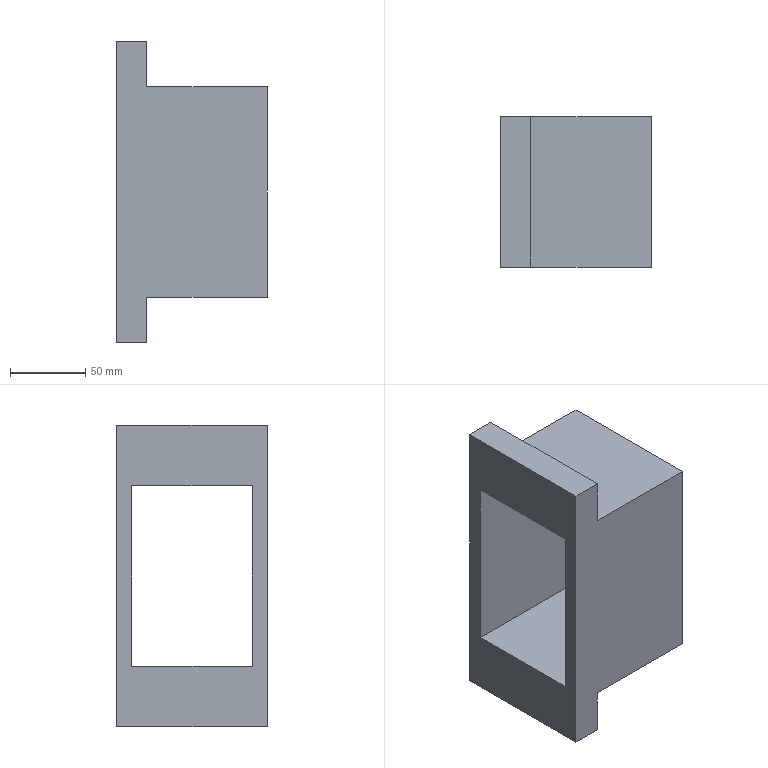Component | SolidWorks | ST60-03-1 | 1 solid | 14 faces | box 100 x 100 x 200 mm | volume 560000 mm3 | plane 14
build123d program:
from build123d import *

# Parameters (mm, degrees)
BOSS_EXTRUDE1_DEPTH = 100
SKETCH2_W           = 120
SKETCH2_H           = 80
CUT_EXTRUDE1_DEPTH  = 207.285


with BuildPart() as part:
    # Sketch1 → Boss-Extrude1 (new body)
    with BuildSketch(Plane.XY):
        Polygon((-19.821, 57.321), (120.179, 57.321), (120.179, -22.679), (150.179, -22.679), (150.179, -42.679), (-49.821, -42.679), (-49.821, -22.679), (-19.821, -22.679), align=None)
    extrude(amount=BOSS_EXTRUDE1_DEPTH)

    # Sketch2 → Cut-Extrude1 (cut, through all)
    with BuildSketch(Plane(origin=(0, 57.321, 0), x_dir=(1, 0, 0), z_dir=(0, 1, 0))):
        with Locations((50.179, -50)):
            Rectangle(SKETCH2_W, SKETCH2_H)
    extrude(amount=-CUT_EXTRUDE1_DEPTH, mode=Mode.SUBTRACT)


solid = part.part

# Placed as in the assembly
solid = solid.moved(Location((-804.328, 45.454, 50.179), (90, 0, -90)))
STEP:
#1=CARTESIAN_POINT('',(-29.41,-2.147,-2.756));
#2=VERTEX_POINT('',#1);
#3=CARTESIAN_POINT('',(-32.559,-2.147,-2.756));
#4=VERTEX_POINT('',#3);
#5=CARTESIAN_POINT('',(-32.559,-2.147,-2.756));
#6=DIRECTION('',(-1.,0.,0.));
#7=VECTOR('',#6,39.37);
#8=LINE('',#5,#7);
#9=EDGE_CURVE('',#2,#4,#8,.T.);
#10=ORIENTED_EDGE('',*,*,#9,.T.);
#11=CARTESIAN_POINT('',(-32.559,1.79,-2.756));
#12=VERTEX_POINT('',#11);
#13=CARTESIAN_POINT('',(-32.559,1.79,-2.756));
#14=DIRECTION('',(-0.,-1.,-0.));
#15=VECTOR('',#14,39.37);
#16=LINE('',#13,#15);
#17=EDGE_CURVE('',#12,#4,#16,.T.);
#18=ORIENTED_EDGE('',*,*,#17,.F.);
#19=CARTESIAN_POINT('',(-29.41,1.79,-2.756));
#20=VERTEX_POINT('',#19);
#21=CARTESIAN_POINT('',(-32.559,1.79,-2.756));
#22=DIRECTION('',(-1.,0.,0.));
#23=VECTOR('',#22,39.37);
#24=LINE('',#21,#23);
#25=EDGE_CURVE('',#20,#12,#24,.T.);
#26=ORIENTED_EDGE('',*,*,#25,.F.);
#27=CARTESIAN_POINT('',(-29.41,1.79,-2.756));
#28=DIRECTION('',(-0.,-1.,-0.));
#29=VECTOR('',#28,39.37);
#30=LINE('',#27,#29);
#31=EDGE_CURVE('',#20,#2,#30,.T.);
#32=ORIENTED_EDGE('',*,*,#31,.T.);
#33=EDGE_LOOP('',(#10,#18,#26,#32));
#34=FACE_OUTER_BOUND('',#33,.T.);
#35=CARTESIAN_POINT('',(-32.559,1.79,-2.756));
#36=DIRECTION('',(0.,-0.,1.));
#37=DIRECTION('',(1.,-0.,-0.));
#38=AXIS2_PLACEMENT_3D('',#35,#36,#37);
#39=PLANE('',#38);
#40=ADVANCED_FACE('',(#34),#39,.F.);
#41=CARTESIAN_POINT('',(-32.559,-2.147,-3.937));
#42=VERTEX_POINT('',#41);
#43=CARTESIAN_POINT('',(-32.559,-2.147,-3.937));
#44=DIRECTION('',(-0.,0.,-1.));
#45=VECTOR('',#44,39.37);
#46=LINE('',#43,#45);
#47=EDGE_CURVE('',#4,#42,#46,.T.);
#48=ORIENTED_EDGE('',*,*,#47,.T.);
#49=CARTESIAN_POINT('',(-32.559,1.79,-3.937));
#50=VERTEX_POINT('',#49);
#51=CARTESIAN_POINT('',(-32.559,1.79,-3.937));
#52=DIRECTION('',(-0.,-1.,-0.));
#53=VECTOR('',#52,39.37);
#54=LINE('',#51,#53);
#55=EDGE_CURVE('',#50,#42,#54,.T.);
#56=ORIENTED_EDGE('',*,*,#55,.F.);
#57=CARTESIAN_POINT('',(-32.559,1.79,-3.937));
#58=DIRECTION('',(-0.,0.,-1.));
#59=VECTOR('',#58,39.37);
#60=LINE('',#57,#59);
#61=EDGE_CURVE('',#12,#50,#60,.T.);
#62=ORIENTED_EDGE('',*,*,#61,.F.);
#63=ORIENTED_EDGE('',*,*,#17,.T.);
#64=EDGE_LOOP('',(#48,#56,#62,#63));
#65=FACE_OUTER_BOUND('',#64,.T.);
#66=CARTESIAN_POINT('',(-32.559,1.79,-3.937));
#67=DIRECTION('',(-1.,0.,0.));
#68=DIRECTION('',(0.,-0.,1.));
#69=AXIS2_PLACEMENT_3D('',#66,#67,#68);
#70=PLANE('',#69);
#71=ADVANCED_FACE('',(#65),#70,.F.);
#72=CARTESIAN_POINT('',(-33.347,-2.147,-3.937));
#73=VERTEX_POINT('',#72);
#74=CARTESIAN_POINT('',(-33.347,-2.147,-3.937));
#75=DIRECTION('',(-1.,0.,-0.));
#76=VECTOR('',#75,39.37);
#77=LINE('',#74,#76);
#78=EDGE_CURVE('',#42,#73,#77,.T.);
#79=ORIENTED_EDGE('',*,*,#78,.T.);
#80=CARTESIAN_POINT('',(-33.347,1.79,-3.937));
#81=VERTEX_POINT('',#80);
#82=CARTESIAN_POINT('',(-33.347,1.79,-3.937));
#83=DIRECTION('',(-0.,-1.,-0.));
#84=VECTOR('',#83,39.37);
#85=LINE('',#82,#84);
#86=EDGE_CURVE('',#81,#73,#85,.T.);
#87=ORIENTED_EDGE('',*,*,#86,.F.);
#88=CARTESIAN_POINT('',(-33.347,1.79,-3.937));
#89=DIRECTION('',(-1.,0.,-0.));
#90=VECTOR('',#89,39.37);
#91=LINE('',#88,#90);
#92=EDGE_CURVE('',#50,#81,#91,.T.);
#93=ORIENTED_EDGE('',*,*,#92,.F.);
#94=ORIENTED_EDGE('',*,*,#55,.T.);
#95=EDGE_LOOP('',(#79,#87,#93,#94));
#96=FACE_OUTER_BOUND('',#95,.T.);
#97=CARTESIAN_POINT('',(-33.347,1.79,-3.937));
#98=DIRECTION('',(-0.,-0.,1.));
#99=DIRECTION('',(-0.,-1.,-0.));
#100=AXIS2_PLACEMENT_3D('',#97,#98,#99);
#101=PLANE('',#100);
#102=ADVANCED_FACE('',(#96),#101,.F.);
#103=CARTESIAN_POINT('',(-33.347,-1.754,2.362));
#104=VERTEX_POINT('',#103);
#105=CARTESIAN_POINT('',(-33.347,-1.754,-2.362));
#106=VERTEX_POINT('',#105);
#107=CARTESIAN_POINT('',(-33.347,-1.754,-2.362));
#108=DIRECTION('',(-0.,0.,-1.));
#109=VECTOR('',#108,39.37);
#110=LINE('',#107,#109);
#111=EDGE_CURVE('',#104,#106,#110,.T.);
#112=ORIENTED_EDGE('',*,*,#111,.T.);
#113=CARTESIAN_POINT('',(-33.347,1.396,-2.362));
#114=VERTEX_POINT('',#113);
#115=CARTESIAN_POINT('',(-33.347,-1.754,-2.362));
#116=DIRECTION('',(0.,1.,0.));
#117=VECTOR('',#116,39.37);
#118=LINE('',#115,#117);
#119=EDGE_CURVE('',#106,#114,#118,.T.);
#120=ORIENTED_EDGE('',*,*,#119,.T.);
#121=CARTESIAN_POINT('',(-33.347,1.396,2.362));
#122=VERTEX_POINT('',#121);
#123=CARTESIAN_POINT('',(-33.347,1.396,-2.362));
#124=DIRECTION('',(0.,-0.,1.));
#125=VECTOR('',#124,39.37);
#126=LINE('',#123,#125);
#127=EDGE_CURVE('',#114,#122,#126,.T.);
#128=ORIENTED_EDGE('',*,*,#127,.T.);
#129=CARTESIAN_POINT('',(-33.347,-1.754,2.362));
#130=DIRECTION('',(-0.,-1.,-0.));
#131=VECTOR('',#130,39.37);
#132=LINE('',#129,#131);
#133=EDGE_CURVE('',#122,#104,#132,.T.);
#134=ORIENTED_EDGE('',*,*,#133,.T.);
#135=EDGE_LOOP('',(#112,#120,#128,#134));
#136=FACE_BOUND('',#135,.T.);
#137=CARTESIAN_POINT('',(-33.347,-2.147,3.937));
#138=VERTEX_POINT('',#137);
#139=CARTESIAN_POINT('',(-33.347,-2.147,3.937));
#140=DIRECTION('',(0.,-0.,1.));
#141=VECTOR('',#140,39.37);
#142=LINE('',#139,#141);
#143=EDGE_CURVE('',#73,#138,#142,.T.);
#144=ORIENTED_EDGE('',*,*,#143,.T.);
#145=CARTESIAN_POINT('',(-33.347,1.79,3.937));
#146=VERTEX_POINT('',#145);
#147=CARTESIAN_POINT('',(-33.347,1.79,3.937));
#148=DIRECTION('',(-0.,-1.,-0.));
#149=VECTOR('',#148,39.37);
#150=LINE('',#147,#149);
#151=EDGE_CURVE('',#146,#138,#150,.T.);
#152=ORIENTED_EDGE('',*,*,#151,.F.);
#153=CARTESIAN_POINT('',(-33.347,1.79,3.937));
#154=DIRECTION('',(0.,-0.,1.));
#155=VECTOR('',#154,39.37);
#156=LINE('',#153,#155);
#157=EDGE_CURVE('',#81,#146,#156,.T.);
#158=ORIENTED_EDGE('',*,*,#157,.F.);
#159=ORIENTED_EDGE('',*,*,#86,.T.);
#160=EDGE_LOOP('',(#144,#152,#158,#159));
#161=FACE_OUTER_BOUND('',#160,.T.);
#162=CARTESIAN_POINT('',(-33.347,1.79,3.937));
#163=DIRECTION('',(1.,-0.,-0.));
#164=DIRECTION('',(-0.,0.,-1.));
#165=AXIS2_PLACEMENT_3D('',#162,#163,#164);
#166=PLANE('',#165);
#167=ADVANCED_FACE('',(#136,#161),#166,.F.);
#168=CARTESIAN_POINT('',(-32.559,-2.147,3.937));
#169=VERTEX_POINT('',#168);
#170=CARTESIAN_POINT('',(-32.559,-2.147,3.937));
#171=DIRECTION('',(1.,-0.,0.));
#172=VECTOR('',#171,39.37);
#173=LINE('',#170,#172);
#174=EDGE_CURVE('',#138,#169,#173,.T.);
#175=ORIENTED_EDGE('',*,*,#174,.T.);
#176=CARTESIAN_POINT('',(-32.559,1.79,3.937));
#177=VERTEX_POINT('',#176);
#178=CARTESIAN_POINT('',(-32.559,1.79,3.937));
#179=DIRECTION('',(-0.,-1.,-0.));
#180=VECTOR('',#179,39.37);
#181=LINE('',#178,#180);
#182=EDGE_CURVE('',#177,#169,#181,.T.);
#183=ORIENTED_EDGE('',*,*,#182,.F.);
#184=CARTESIAN_POINT('',(-32.559,1.79,3.937));
#185=DIRECTION('',(1.,-0.,0.));
#186=VECTOR('',#185,39.37);
#187=LINE('',#184,#186);
#188=EDGE_CURVE('',#146,#177,#187,.T.);
#189=ORIENTED_EDGE('',*,*,#188,.F.);
#190=ORIENTED_EDGE('',*,*,#151,.T.);
#191=EDGE_LOOP('',(#175,#183,#189,#190));
#192=FACE_OUTER_BOUND('',#191,.T.);
#193=CARTESIAN_POINT('',(-32.559,1.79,3.937));
#194=DIRECTION('',(0.,0.,-1.));
#195=DIRECTION('',(0.,1.,0.));
#196=AXIS2_PLACEMENT_3D('',#193,#194,#195);
#197=PLANE('',#196);
#198=ADVANCED_FACE('',(#192),#197,.F.);
#199=CARTESIAN_POINT('',(-32.559,-2.147,2.756));
#200=VERTEX_POINT('',#199);
#201=CARTESIAN_POINT('',(-32.559,-2.147,2.756));
#202=DIRECTION('',(-0.,0.,-1.));
#203=VECTOR('',#202,39.37);
#204=LINE('',#201,#203);
#205=EDGE_CURVE('',#169,#200,#204,.T.);
#206=ORIENTED_EDGE('',*,*,#205,.T.);
#207=CARTESIAN_POINT('',(-32.559,1.79,2.756));
#208=VERTEX_POINT('',#207);
#209=CARTESIAN_POINT('',(-32.559,1.79,2.756));
#210=DIRECTION('',(-0.,-1.,-0.));
#211=VECTOR('',#210,39.37);
#212=LINE('',#209,#211);
#213=EDGE_CURVE('',#208,#200,#212,.T.);
#214=ORIENTED_EDGE('',*,*,#213,.F.);
#215=CARTESIAN_POINT('',(-32.559,1.79,2.756));
#216=DIRECTION('',(-0.,0.,-1.));
#217=VECTOR('',#216,39.37);
#218=LINE('',#215,#217);
#219=EDGE_CURVE('',#177,#208,#218,.T.);
#220=ORIENTED_EDGE('',*,*,#219,.F.);
#221=ORIENTED_EDGE('',*,*,#182,.T.);
#222=EDGE_LOOP('',(#206,#214,#220,#221));
#223=FACE_OUTER_BOUND('',#222,.T.);
#224=CARTESIAN_POINT('',(-32.559,1.79,2.756));
#225=DIRECTION('',(-1.,0.,0.));
#226=DIRECTION('',(0.,-0.,1.));
#227=AXIS2_PLACEMENT_3D('',#224,#225,#226);
#228=PLANE('',#227);
#229=ADVANCED_FACE('',(#223),#228,.F.);
#230=CARTESIAN_POINT('',(-29.41,-2.147,2.756));
#231=VERTEX_POINT('',#230);
#232=CARTESIAN_POINT('',(-29.41,-2.147,2.756));
#233=DIRECTION('',(1.,-0.,-0.));
#234=VECTOR('',#233,39.37);
#235=LINE('',#232,#234);
#236=EDGE_CURVE('',#200,#231,#235,.T.);
#237=ORIENTED_EDGE('',*,*,#236,.T.);
#238=CARTESIAN_POINT('',(-29.41,1.79,2.756));
#239=VERTEX_POINT('',#238);
#240=CARTESIAN_POINT('',(-29.41,1.79,2.756));
#241=DIRECTION('',(-0.,-1.,-0.));
#242=VECTOR('',#241,39.37);
#243=LINE('',#240,#242);
#244=EDGE_CURVE('',#239,#231,#243,.T.);
#245=ORIENTED_EDGE('',*,*,#244,.F.);
#246=CARTESIAN_POINT('',(-29.41,1.79,2.756));
#247=DIRECTION('',(1.,-0.,-0.));
#248=VECTOR('',#247,39.37);
#249=LINE('',#246,#248);
#250=EDGE_CURVE('',#208,#239,#249,.T.);
#251=ORIENTED_EDGE('',*,*,#250,.F.);
#252=ORIENTED_EDGE('',*,*,#213,.T.);
#253=EDGE_LOOP('',(#237,#245,#251,#252));
#254=FACE_OUTER_BOUND('',#253,.T.);
#255=CARTESIAN_POINT('',(-29.41,1.79,2.756));
#256=DIRECTION('',(-0.,0.,-1.));
#257=DIRECTION('',(-1.,0.,0.));
#258=AXIS2_PLACEMENT_3D('',#255,#256,#257);
#259=PLANE('',#258);
#260=ADVANCED_FACE('',(#254),#259,.F.);
#261=CARTESIAN_POINT('',(-29.41,1.396,-2.362));
#262=VERTEX_POINT('',#261);
#263=CARTESIAN_POINT('',(-29.41,1.396,2.362));
#264=VERTEX_POINT('',#263);
#265=CARTESIAN_POINT('',(-29.41,1.396,-2.362));
#266=DIRECTION('',(0.,-0.,1.));
#267=VECTOR('',#266,39.37);
#268=LINE('',#265,#267);
#269=EDGE_CURVE('',#262,#264,#268,.T.);
#270=ORIENTED_EDGE('',*,*,#269,.F.);
#271=CARTESIAN_POINT('',(-29.41,-1.754,-2.362));
#272=VERTEX_POINT('',#271);
#273=CARTESIAN_POINT('',(-29.41,-1.754,-2.362));
#274=DIRECTION('',(0.,1.,0.));
#275=VECTOR('',#274,39.37);
#276=LINE('',#273,#275);
#277=EDGE_CURVE('',#272,#262,#276,.T.);
#278=ORIENTED_EDGE('',*,*,#277,.F.);
#279=CARTESIAN_POINT('',(-29.41,-1.754,2.362));
#280=VERTEX_POINT('',#279);
#281=CARTESIAN_POINT('',(-29.41,-1.754,-2.362));
#282=DIRECTION('',(-0.,0.,-1.));
#283=VECTOR('',#282,39.37);
#284=LINE('',#281,#283);
#285=EDGE_CURVE('',#280,#272,#284,.T.);
#286=ORIENTED_EDGE('',*,*,#285,.F.);
#287=CARTESIAN_POINT('',(-29.41,-1.754,2.362));
#288=DIRECTION('',(-0.,-1.,-0.));
#289=VECTOR('',#288,39.37);
#290=LINE('',#287,#289);
#291=EDGE_CURVE('',#264,#280,#290,.T.);
#292=ORIENTED_EDGE('',*,*,#291,.F.);
#293=EDGE_LOOP('',(#270,#278,#286,#292));
#294=FACE_BOUND('',#293,.T.);
#295=CARTESIAN_POINT('',(-29.41,-2.147,-2.756));
#296=DIRECTION('',(-0.,0.,-1.));
#297=VECTOR('',#296,39.37);
#298=LINE('',#295,#297);
#299=EDGE_CURVE('',#231,#2,#298,.T.);
#300=ORIENTED_EDGE('',*,*,#299,.T.);
#301=ORIENTED_EDGE('',*,*,#31,.F.);
#302=CARTESIAN_POINT('',(-29.41,1.79,-2.756));
#303=DIRECTION('',(-0.,0.,-1.));
#304=VECTOR('',#303,39.37);
#305=LINE('',#302,#304);
#306=EDGE_CURVE('',#239,#20,#305,.T.);
#307=ORIENTED_EDGE('',*,*,#306,.F.);
#308=ORIENTED_EDGE('',*,*,#244,.T.);
#309=EDGE_LOOP('',(#300,#301,#307,#308));
#310=FACE_OUTER_BOUND('',#309,.T.);
#311=CARTESIAN_POINT('',(-29.41,1.79,-2.756));
#312=DIRECTION('',(-1.,0.,0.));
#313=DIRECTION('',(0.,-0.,1.));
#314=AXIS2_PLACEMENT_3D('',#311,#312,#313);
#315=PLANE('',#314);
#316=ADVANCED_FACE('',(#294,#310),#315,.F.);
#317=ORIENTED_EDGE('',*,*,#25,.T.);
#318=ORIENTED_EDGE('',*,*,#61,.T.);
#319=ORIENTED_EDGE('',*,*,#92,.T.);
#320=ORIENTED_EDGE('',*,*,#157,.T.);
#321=ORIENTED_EDGE('',*,*,#188,.T.);
#322=ORIENTED_EDGE('',*,*,#219,.T.);
#323=ORIENTED_EDGE('',*,*,#250,.T.);
#324=ORIENTED_EDGE('',*,*,#306,.T.);
#325=EDGE_LOOP('',(#317,#318,#319,#320,#321,#322,#323,#324));
#326=FACE_OUTER_BOUND('',#325,.T.);
#327=CARTESIAN_POINT('',(-31.666,1.79,-1.976));
#328=DIRECTION('',(-0.,-1.,-0.));
#329=DIRECTION('',(0.,0.,-1.));
#330=AXIS2_PLACEMENT_3D('',#327,#328,#329);
#331=PLANE('',#330);
#332=ADVANCED_FACE('',(#326),#331,.F.);
#333=ORIENTED_EDGE('',*,*,#9,.F.);
#334=ORIENTED_EDGE('',*,*,#299,.F.);
#335=ORIENTED_EDGE('',*,*,#236,.F.);
#336=ORIENTED_EDGE('',*,*,#205,.F.);
#337=ORIENTED_EDGE('',*,*,#174,.F.);
#338=ORIENTED_EDGE('',*,*,#143,.F.);
#339=ORIENTED_EDGE('',*,*,#78,.F.);
#340=ORIENTED_EDGE('',*,*,#47,.F.);
#341=EDGE_LOOP('',(#333,#334,#335,#336,#337,#338,#339,#340));
#342=FACE_OUTER_BOUND('',#341,.T.);
#343=CARTESIAN_POINT('',(-31.666,-2.147,-1.976));
#344=DIRECTION('',(-0.,-1.,-0.));
#345=DIRECTION('',(0.,0.,-1.));
#346=AXIS2_PLACEMENT_3D('',#343,#344,#345);
#347=PLANE('',#346);
#348=ADVANCED_FACE('',(#342),#347,.T.);
#349=ORIENTED_EDGE('',*,*,#277,.T.);
#350=CARTESIAN_POINT('',(-33.347,1.396,-2.362));
#351=DIRECTION('',(1.,-0.,-0.));
#352=VECTOR('',#351,39.37);
#353=LINE('',#350,#352);
#354=EDGE_CURVE('',#114,#262,#353,.T.);
#355=ORIENTED_EDGE('',*,*,#354,.F.);
#356=ORIENTED_EDGE('',*,*,#119,.F.);
#357=CARTESIAN_POINT('',(-33.347,-1.754,-2.362));
#358=DIRECTION('',(1.,-0.,-0.));
#359=VECTOR('',#358,39.37);
#360=LINE('',#357,#359);
#361=EDGE_CURVE('',#106,#272,#360,.T.);
#362=ORIENTED_EDGE('',*,*,#361,.T.);
#363=EDGE_LOOP('',(#349,#355,#356,#362));
#364=FACE_OUTER_BOUND('',#363,.T.);
#365=CARTESIAN_POINT('',(-33.347,-1.754,-2.362));
#366=DIRECTION('',(-0.,0.,-1.));
#367=DIRECTION('',(0.,1.,0.));
#368=AXIS2_PLACEMENT_3D('',#365,#366,#367);
#369=PLANE('',#368);
#370=ADVANCED_FACE('',(#364),#369,.F.);
#371=ORIENTED_EDGE('',*,*,#285,.T.);
#372=ORIENTED_EDGE('',*,*,#361,.F.);
#373=ORIENTED_EDGE('',*,*,#111,.F.);
#374=CARTESIAN_POINT('',(-33.347,-1.754,2.362));
#375=DIRECTION('',(1.,-0.,-0.));
#376=VECTOR('',#375,39.37);
#377=LINE('',#374,#376);
#378=EDGE_CURVE('',#104,#280,#377,.T.);
#379=ORIENTED_EDGE('',*,*,#378,.T.);
#380=EDGE_LOOP('',(#371,#372,#373,#379));
#381=FACE_OUTER_BOUND('',#380,.T.);
#382=CARTESIAN_POINT('',(-33.347,-1.754,-2.362));
#383=DIRECTION('',(-0.,-1.,-0.));
#384=DIRECTION('',(0.,0.,-1.));
#385=AXIS2_PLACEMENT_3D('',#382,#383,#384);
#386=PLANE('',#385);
#387=ADVANCED_FACE('',(#381),#386,.F.);
#388=ORIENTED_EDGE('',*,*,#291,.T.);
#389=ORIENTED_EDGE('',*,*,#378,.F.);
#390=ORIENTED_EDGE('',*,*,#133,.F.);
#391=CARTESIAN_POINT('',(-33.347,1.396,2.362));
#392=DIRECTION('',(1.,-0.,-0.));
#393=VECTOR('',#392,39.37);
#394=LINE('',#391,#393);
#395=EDGE_CURVE('',#122,#264,#394,.T.);
#396=ORIENTED_EDGE('',*,*,#395,.T.);
#397=EDGE_LOOP('',(#388,#389,#390,#396));
#398=FACE_OUTER_BOUND('',#397,.T.);
#399=CARTESIAN_POINT('',(-33.347,-1.754,2.362));
#400=DIRECTION('',(0.,-0.,1.));
#401=DIRECTION('',(1.,-0.,-0.));
#402=AXIS2_PLACEMENT_3D('',#399,#400,#401);
#403=PLANE('',#402);
#404=ADVANCED_FACE('',(#398),#403,.F.);
#405=ORIENTED_EDGE('',*,*,#269,.T.);
#406=ORIENTED_EDGE('',*,*,#395,.F.);
#407=ORIENTED_EDGE('',*,*,#127,.F.);
#408=ORIENTED_EDGE('',*,*,#354,.T.);
#409=EDGE_LOOP('',(#405,#406,#407,#408));
#410=FACE_OUTER_BOUND('',#409,.T.);
#411=CARTESIAN_POINT('',(-33.347,1.396,-2.362));
#412=DIRECTION('',(0.,1.,0.));
#413=DIRECTION('',(-0.,-0.,1.));
#414=AXIS2_PLACEMENT_3D('',#411,#412,#413);
#415=PLANE('',#414);
#416=ADVANCED_FACE('',(#410),#415,.F.);
#417=CLOSED_SHELL('',(#40,#71,#102,#167,#198,#229,#260,#316,#332,#348,#370,#387,#404,#416));
#418=MANIFOLD_SOLID_BREP('',#417);
#419=CARTESIAN_POINT('',(0.,0.,0.));
#420=DIRECTION('',(0.,0.,1.));
#421=DIRECTION('',(1.,0.,0.));
#422=AXIS2_PLACEMENT_3D('',#419,#420,#421);
#423=(LENGTH_UNIT()NAMED_UNIT(*)SI_UNIT($,.METRE.));
#424=LENGTH_MEASURE_WITH_UNIT(LENGTH_MEASURE(0.0254),#423);
#425=DIMENSIONAL_EXPONENTS(1.,0.,0.,0.,0.,0.,0.);
#426=(CONVERSION_BASED_UNIT('',#424)LENGTH_UNIT()NAMED_UNIT(#425));
#427=UNCERTAINTY_MEASURE_WITH_UNIT(LENGTH_MEASURE(0.00001),#426,'','');
#428=(NAMED_UNIT(*)PLANE_ANGLE_UNIT()SI_UNIT($,.RADIAN.));
#429=(NAMED_UNIT(*)SI_UNIT($,.STERADIAN.)SOLID_ANGLE_UNIT());
#430=(GEOMETRIC_REPRESENTATION_CONTEXT(3)GLOBAL_UNCERTAINTY_ASSIGNED_CONTEXT((#427))GLOBAL_UNIT_ASSIGNED_CONTEXT((#426,#428,#429))REPRESENTATION_CONTEXT('',''));
#431=ADVANCED_BREP_SHAPE_REPRESENTATION('',(#418,#422),#430);
#432=COLOUR_RGB('',0.7922,0.8196,0.9333);
#433=FILL_AREA_STYLE_COLOUR('',#432);
#434=FILL_AREA_STYLE('',(#433));
#435=SURFACE_STYLE_FILL_AREA(#434);
#436=SURFACE_SIDE_STYLE('',(#435));
#437=SURFACE_STYLE_USAGE(.BOTH.,#436);
#438=PRESENTATION_STYLE_ASSIGNMENT((#437));
#439=STYLED_ITEM('',(#438),#418);
#440=(LENGTH_UNIT()NAMED_UNIT(*)SI_UNIT($,.METRE.));
#441=LENGTH_MEASURE_WITH_UNIT(LENGTH_MEASURE(0.0254),#440);
#442=DIMENSIONAL_EXPONENTS(1.,0.,0.,0.,0.,0.,0.);
#443=(CONVERSION_BASED_UNIT('',#441)LENGTH_UNIT()NAMED_UNIT(#442));
#444=UNCERTAINTY_MEASURE_WITH_UNIT(LENGTH_MEASURE(0.00001),#443,'','');
#445=(NAMED_UNIT(*)PLANE_ANGLE_UNIT()SI_UNIT($,.RADIAN.));
#446=(NAMED_UNIT(*)SI_UNIT($,.STERADIAN.)SOLID_ANGLE_UNIT());
#447=(GEOMETRIC_REPRESENTATION_CONTEXT(3)GLOBAL_UNCERTAINTY_ASSIGNED_CONTEXT((#444))GLOBAL_UNIT_ASSIGNED_CONTEXT((#443,#445,#446))REPRESENTATION_CONTEXT('',''));
#448=MECHANICAL_DESIGN_GEOMETRIC_PRESENTATION_REPRESENTATION('',(#439),#447);
#449=PRESENTATION_LAYER_ASSIGNMENT('','',(#439));